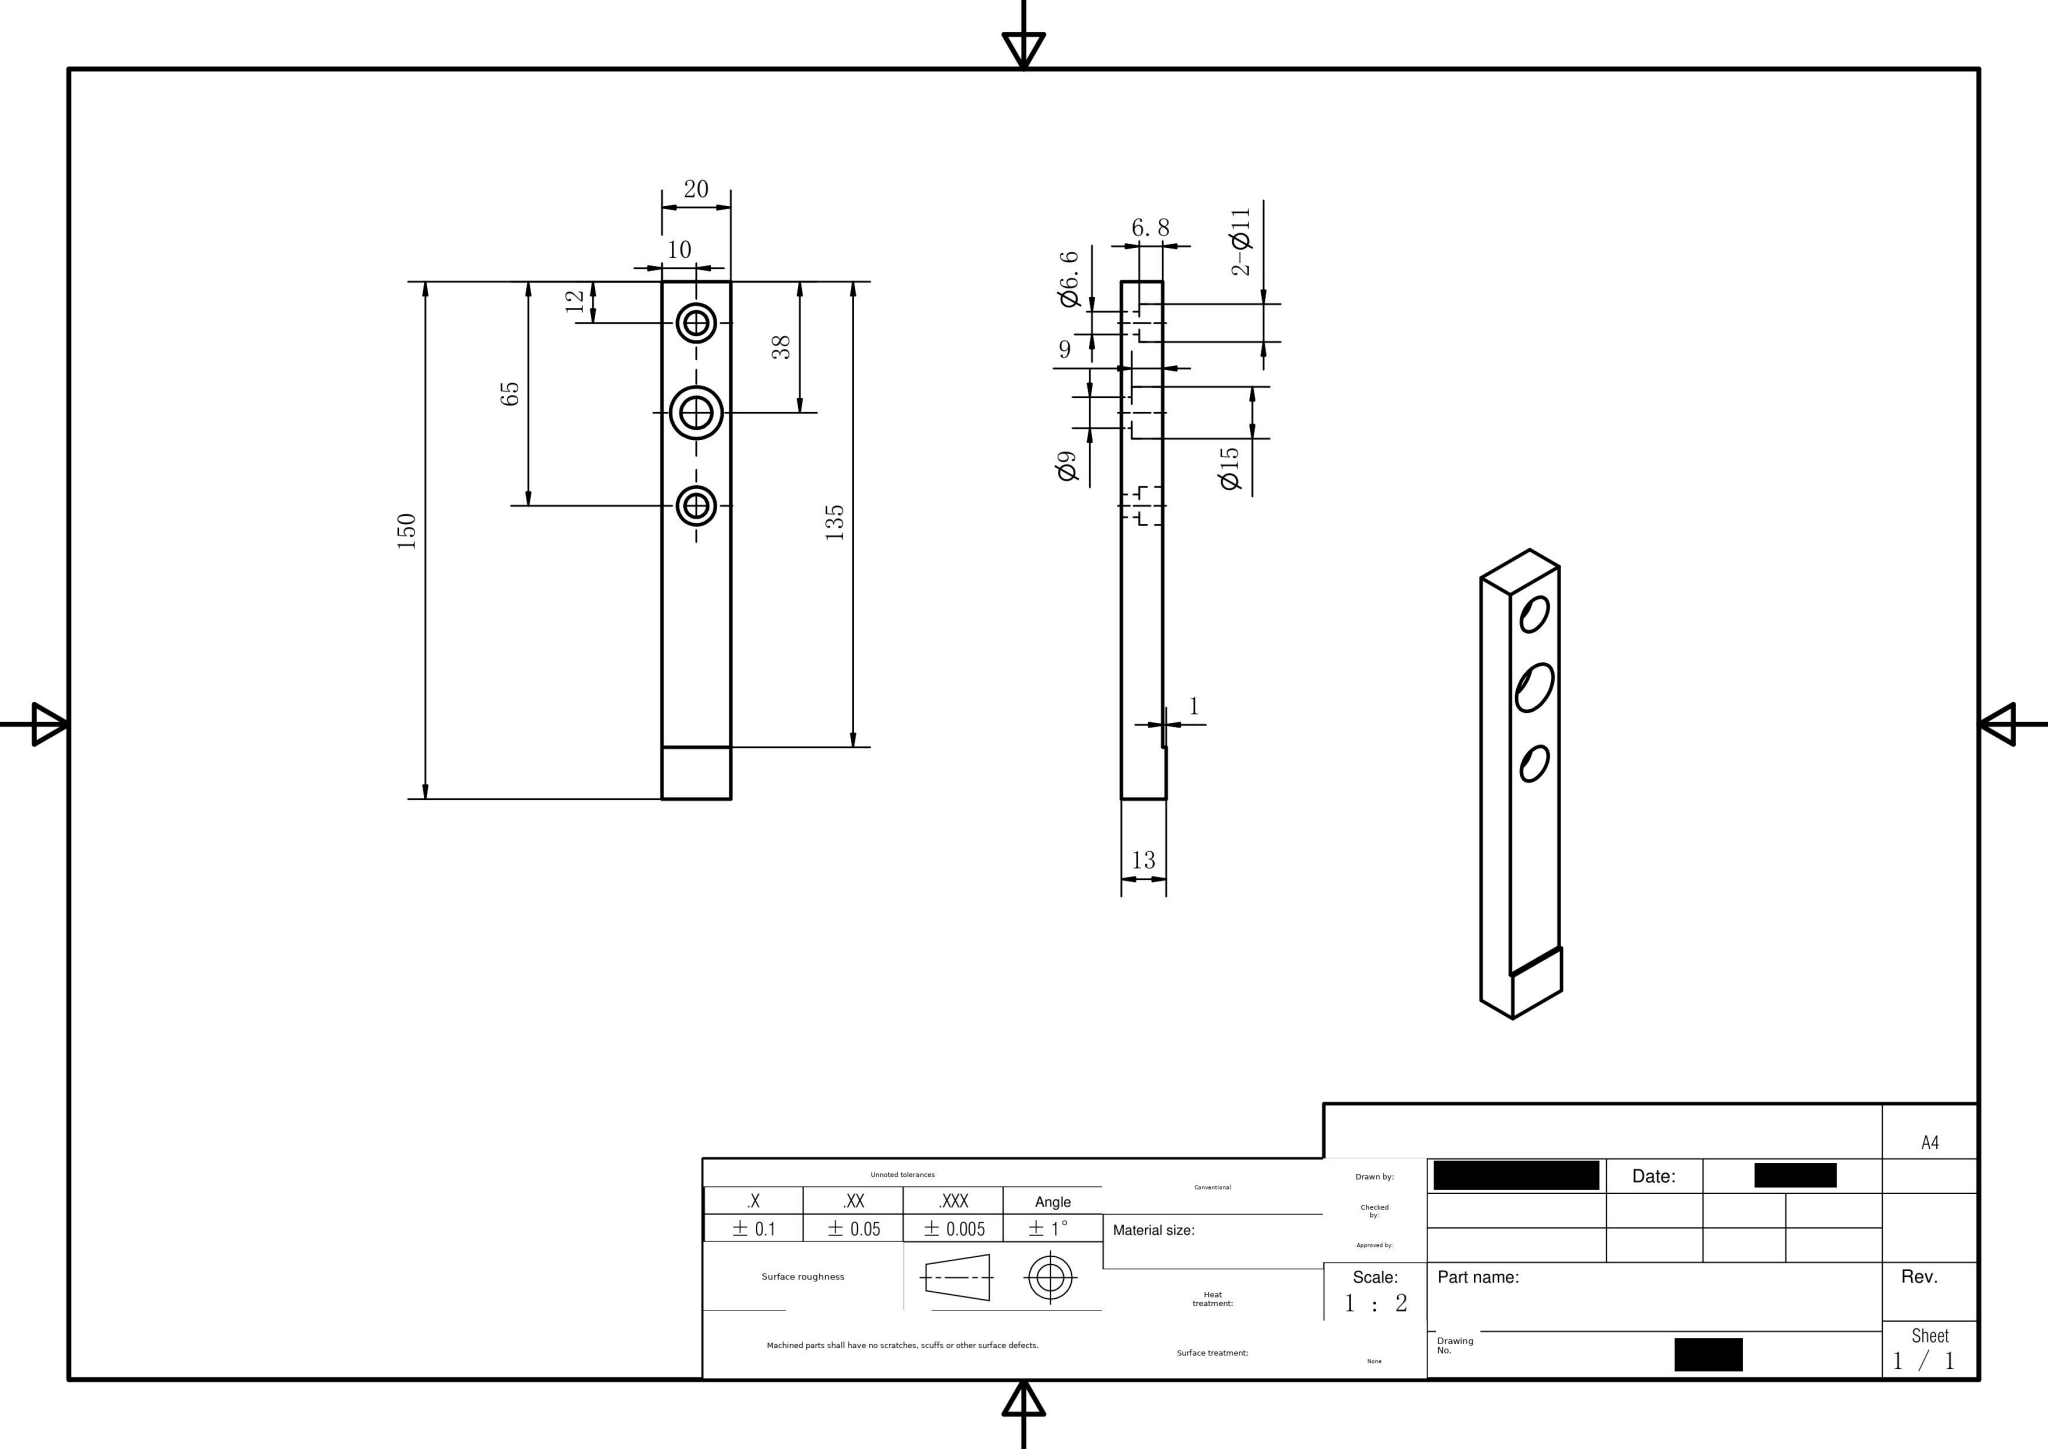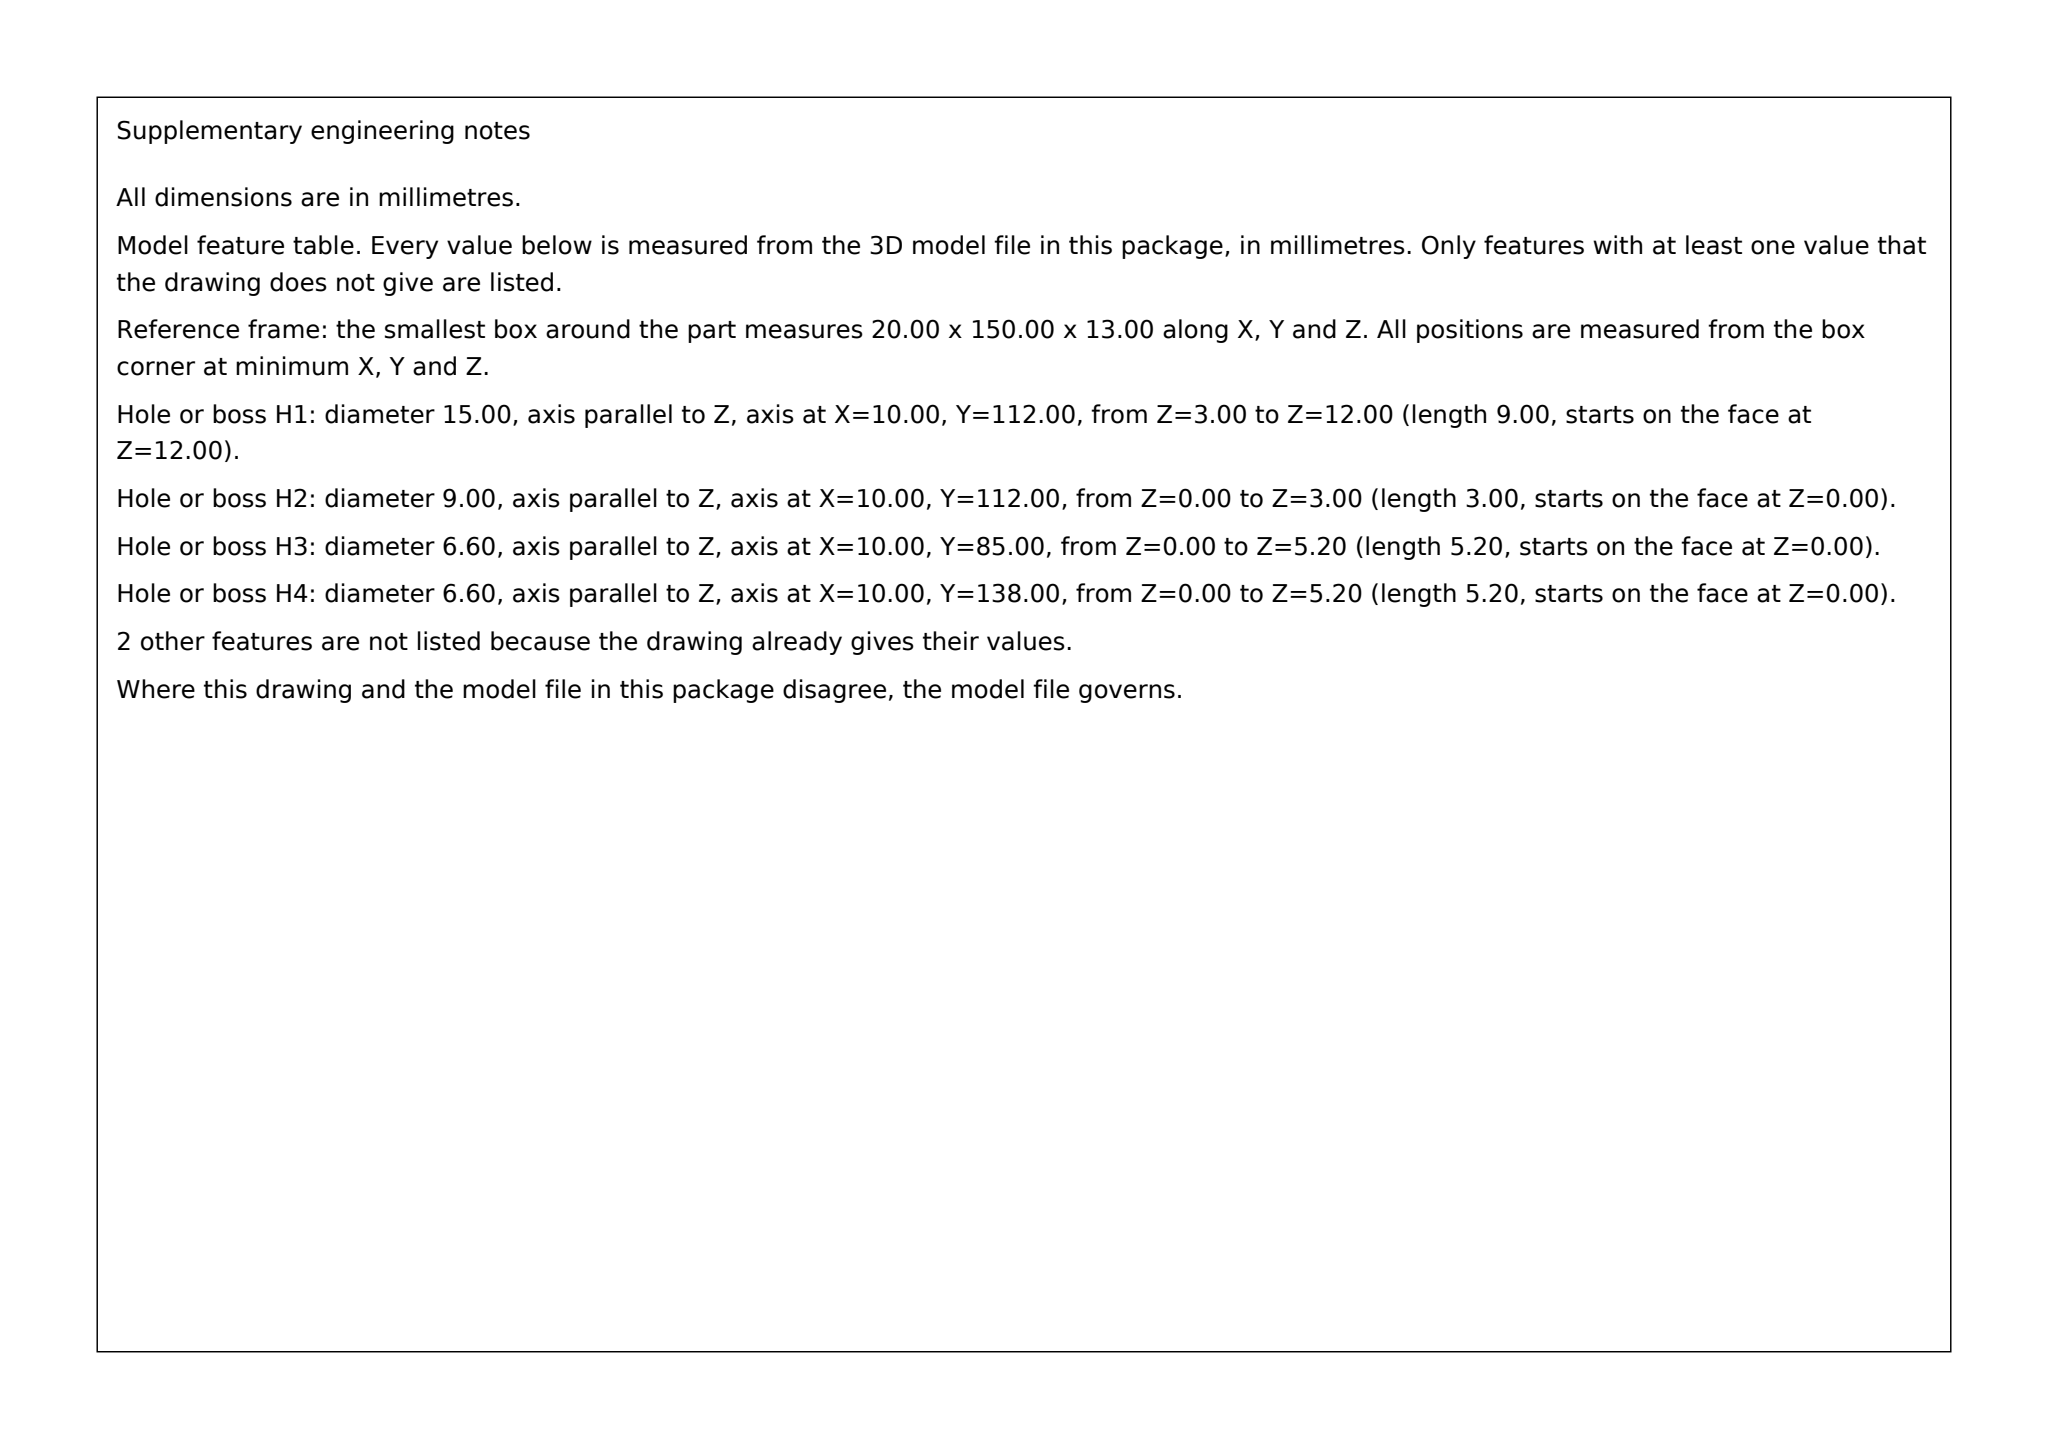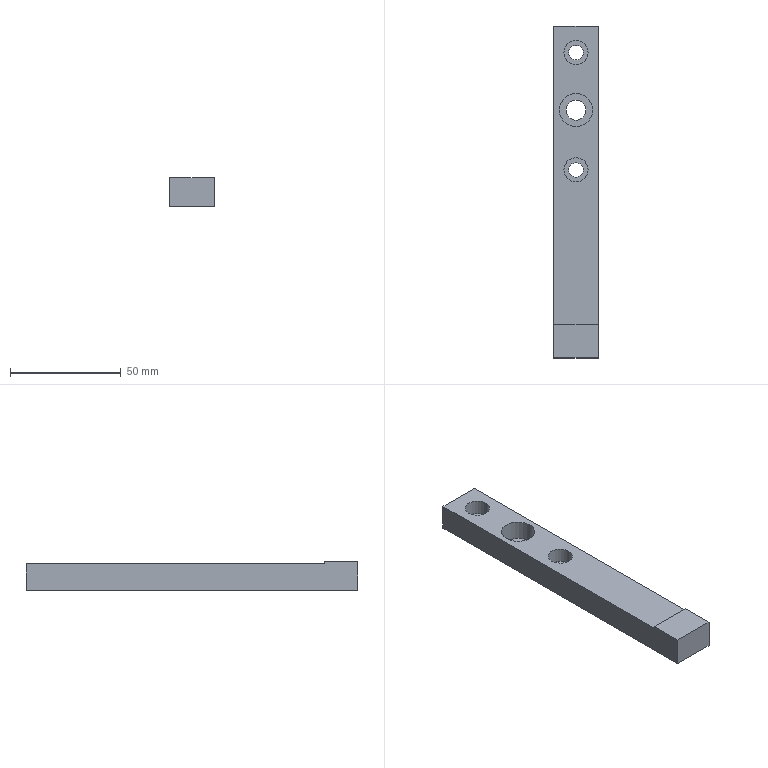Part | SolidWorks | mm | 1 solid | 23 faces | box 20 x 150 x 13 mm | volume 32870 mm3 | cylinder 12 | plane 11 | commonest cylinder face diameters 11 x4 6.6 x4 15 x2 9 x2
build123d program:
from build123d import *

# Parameters (mm, degrees)
SKETCH1_W                                  = 20
SKETCH1_H                                  = 150
BOSS_EXTRUDE1_DEPTH                        = 13
SKETCH2_W                                  = 1
SKETCH2_H                                  = 135
CUT_EXTRUDE1_DEPTH                         = 79.702
M6_HEX_HEAD_BOLT_COUNTERBORE_1_D           = 6.6
M6_HEX_HEAD_BOLT_COUNTERBORE_1_CBORE_D     = 11
M6_HEX_HEAD_BOLT_COUNTERBORE_1_CBORE_DEPTH = 6.8
M8_HEX_HEAD_BOLT_COUNTERBORE_1_D           = 9
M8_HEX_HEAD_BOLT_COUNTERBORE_1_CBORE_D     = 15
M8_HEX_HEAD_BOLT_COUNTERBORE_1_CBORE_DEPTH = 9


with BuildPart() as part:
    # Sketch1 → Boss-Extrude1 (new body)
    with BuildSketch(Plane.XY.offset(13)):
        Rectangle(SKETCH1_W, SKETCH1_H)
    extrude(amount=-BOSS_EXTRUDE1_DEPTH)

    # Sketch2 → Cut-Extrude1 (cut, through all)
    with BuildSketch(Plane(origin=(10, 0, 0), x_dir=(0, 0, -1), z_dir=(1, 0, 0))):
        with Locations((-12.5, 7.5)):
            Rectangle(SKETCH2_W, SKETCH2_H)
    extrude(amount=-CUT_EXTRUDE1_DEPTH, mode=Mode.SUBTRACT)

    # M6 Hex Head Bolt Counterbore 1 (through all)
    with Locations(Plane.XY.offset(12)):
        with Locations((0, 63), (0, 10)):
            CounterBoreHole(M6_HEX_HEAD_BOLT_COUNTERBORE_1_D / 2, M6_HEX_HEAD_BOLT_COUNTERBORE_1_CBORE_D / 2, M6_HEX_HEAD_BOLT_COUNTERBORE_1_CBORE_DEPTH)

    # M8 Hex Head Bolt Counterbore 1 (through all)
    with Locations(Plane.XY.offset(12)):
        with Locations((0, 37)):
            CounterBoreHole(M8_HEX_HEAD_BOLT_COUNTERBORE_1_D / 2, M8_HEX_HEAD_BOLT_COUNTERBORE_1_CBORE_D / 2, M8_HEX_HEAD_BOLT_COUNTERBORE_1_CBORE_DEPTH)


solid = part.part
STEP:
#1=CARTESIAN_POINT('',(-7.5,37.,3.));
#2=VERTEX_POINT('',#1);
#3=CARTESIAN_POINT('',(7.5,37.,3.));
#4=VERTEX_POINT('',#3);
#5=CARTESIAN_POINT('',(0.,37.,3.));
#6=DIRECTION('',(0.,0.,1.));
#7=DIRECTION('',(1.,0.,0.));
#8=AXIS2_PLACEMENT_3D('',#5,#6,#7);
#9=CIRCLE('',#8,7.5);
#10=EDGE_CURVE('',#2,#4,#9,.T.);
#11=ORIENTED_EDGE('',*,*,#10,.F.);
#12=CARTESIAN_POINT('',(-7.5,37.,12.));
#13=VERTEX_POINT('',#12);
#14=CARTESIAN_POINT('',(-7.5,37.,12.));
#15=DIRECTION('',(0.,0.,1.));
#16=VECTOR('',#15,1000.);
#17=LINE('',#14,#16);
#18=EDGE_CURVE('',#2,#13,#17,.T.);
#19=ORIENTED_EDGE('',*,*,#18,.T.);
#20=CARTESIAN_POINT('',(7.5,37.,12.));
#21=VERTEX_POINT('',#20);
#22=CARTESIAN_POINT('',(0.,37.,12.));
#23=DIRECTION('',(0.,0.,1.));
#24=DIRECTION('',(1.,0.,0.));
#25=AXIS2_PLACEMENT_3D('',#22,#23,#24);
#26=CIRCLE('',#25,7.5);
#27=EDGE_CURVE('',#13,#21,#26,.T.);
#28=ORIENTED_EDGE('',*,*,#27,.T.);
#29=CARTESIAN_POINT('',(7.5,37.,12.));
#30=DIRECTION('',(0.,0.,1.));
#31=VECTOR('',#30,1000.);
#32=LINE('',#29,#31);
#33=EDGE_CURVE('',#4,#21,#32,.T.);
#34=ORIENTED_EDGE('',*,*,#33,.F.);
#35=EDGE_LOOP('',(#11,#19,#28,#34));
#36=FACE_OUTER_BOUND('',#35,.T.);
#37=CARTESIAN_POINT('',(0.,37.,12.));
#38=DIRECTION('',(0.,0.,1.));
#39=DIRECTION('',(1.,0.,0.));
#40=AXIS2_PLACEMENT_3D('',#37,#38,#39);
#41=CYLINDRICAL_SURFACE('',#40,7.5);
#42=ADVANCED_FACE('',(#36),#41,.F.);
#43=CARTESIAN_POINT('',(-4.5,37.,0.));
#44=VERTEX_POINT('',#43);
#45=CARTESIAN_POINT('',(4.5,37.,0.));
#46=VERTEX_POINT('',#45);
#47=CARTESIAN_POINT('',(0.,37.,0.));
#48=DIRECTION('',(0.,0.,1.));
#49=DIRECTION('',(1.,0.,0.));
#50=AXIS2_PLACEMENT_3D('',#47,#48,#49);
#51=CIRCLE('',#50,4.5);
#52=EDGE_CURVE('',#44,#46,#51,.T.);
#53=ORIENTED_EDGE('',*,*,#52,.F.);
#54=CARTESIAN_POINT('',(-4.5,37.,3.));
#55=VERTEX_POINT('',#54);
#56=CARTESIAN_POINT('',(-4.5,37.,12.));
#57=DIRECTION('',(0.,0.,1.));
#58=VECTOR('',#57,1000.);
#59=LINE('',#56,#58);
#60=EDGE_CURVE('',#44,#55,#59,.T.);
#61=ORIENTED_EDGE('',*,*,#60,.T.);
#62=CARTESIAN_POINT('',(4.5,37.,3.));
#63=VERTEX_POINT('',#62);
#64=CARTESIAN_POINT('',(0.,37.,3.));
#65=DIRECTION('',(0.,0.,1.));
#66=DIRECTION('',(1.,0.,0.));
#67=AXIS2_PLACEMENT_3D('',#64,#65,#66);
#68=CIRCLE('',#67,4.5);
#69=EDGE_CURVE('',#55,#63,#68,.T.);
#70=ORIENTED_EDGE('',*,*,#69,.T.);
#71=CARTESIAN_POINT('',(4.5,37.,12.));
#72=DIRECTION('',(0.,0.,1.));
#73=VECTOR('',#72,1000.);
#74=LINE('',#71,#73);
#75=EDGE_CURVE('',#46,#63,#74,.T.);
#76=ORIENTED_EDGE('',*,*,#75,.F.);
#77=EDGE_LOOP('',(#53,#61,#70,#76));
#78=FACE_OUTER_BOUND('',#77,.T.);
#79=CARTESIAN_POINT('',(0.,37.,12.));
#80=DIRECTION('',(0.,0.,1.));
#81=DIRECTION('',(1.,0.,0.));
#82=AXIS2_PLACEMENT_3D('',#79,#80,#81);
#83=CYLINDRICAL_SURFACE('',#82,4.5);
#84=ADVANCED_FACE('',(#78),#83,.F.);
#85=CARTESIAN_POINT('',(-5.5,63.,5.2));
#86=VERTEX_POINT('',#85);
#87=CARTESIAN_POINT('',(5.5,63.,5.2));
#88=VERTEX_POINT('',#87);
#89=CARTESIAN_POINT('',(0.,63.,5.2));
#90=DIRECTION('',(0.,0.,1.));
#91=DIRECTION('',(1.,0.,0.));
#92=AXIS2_PLACEMENT_3D('',#89,#90,#91);
#93=CIRCLE('',#92,5.5);
#94=EDGE_CURVE('',#86,#88,#93,.T.);
#95=ORIENTED_EDGE('',*,*,#94,.F.);
#96=CARTESIAN_POINT('',(-5.5,63.,12.));
#97=VERTEX_POINT('',#96);
#98=CARTESIAN_POINT('',(-5.5,63.,12.));
#99=DIRECTION('',(0.,0.,1.));
#100=VECTOR('',#99,1000.);
#101=LINE('',#98,#100);
#102=EDGE_CURVE('',#86,#97,#101,.T.);
#103=ORIENTED_EDGE('',*,*,#102,.T.);
#104=CARTESIAN_POINT('',(5.5,63.,12.));
#105=VERTEX_POINT('',#104);
#106=CARTESIAN_POINT('',(0.,63.,12.));
#107=DIRECTION('',(0.,0.,1.));
#108=DIRECTION('',(1.,0.,0.));
#109=AXIS2_PLACEMENT_3D('',#106,#107,#108);
#110=CIRCLE('',#109,5.5);
#111=EDGE_CURVE('',#97,#105,#110,.T.);
#112=ORIENTED_EDGE('',*,*,#111,.T.);
#113=CARTESIAN_POINT('',(5.5,63.,12.));
#114=DIRECTION('',(0.,0.,1.));
#115=VECTOR('',#114,1000.);
#116=LINE('',#113,#115);
#117=EDGE_CURVE('',#88,#105,#116,.T.);
#118=ORIENTED_EDGE('',*,*,#117,.F.);
#119=EDGE_LOOP('',(#95,#103,#112,#118));
#120=FACE_OUTER_BOUND('',#119,.T.);
#121=CARTESIAN_POINT('',(0.,63.,12.));
#122=DIRECTION('',(0.,0.,1.));
#123=DIRECTION('',(1.,0.,0.));
#124=AXIS2_PLACEMENT_3D('',#121,#122,#123);
#125=CYLINDRICAL_SURFACE('',#124,5.5);
#126=ADVANCED_FACE('',(#120),#125,.F.);
#127=CARTESIAN_POINT('',(-3.3,63.,0.));
#128=VERTEX_POINT('',#127);
#129=CARTESIAN_POINT('',(3.3,63.,0.));
#130=VERTEX_POINT('',#129);
#131=CARTESIAN_POINT('',(0.,63.,0.));
#132=DIRECTION('',(0.,0.,1.));
#133=DIRECTION('',(1.,0.,0.));
#134=AXIS2_PLACEMENT_3D('',#131,#132,#133);
#135=CIRCLE('',#134,3.3);
#136=EDGE_CURVE('',#128,#130,#135,.T.);
#137=ORIENTED_EDGE('',*,*,#136,.F.);
#138=CARTESIAN_POINT('',(-3.3,63.,5.2));
#139=VERTEX_POINT('',#138);
#140=CARTESIAN_POINT('',(-3.3,63.,12.));
#141=DIRECTION('',(0.,0.,1.));
#142=VECTOR('',#141,1000.);
#143=LINE('',#140,#142);
#144=EDGE_CURVE('',#128,#139,#143,.T.);
#145=ORIENTED_EDGE('',*,*,#144,.T.);
#146=CARTESIAN_POINT('',(3.3,63.,5.2));
#147=VERTEX_POINT('',#146);
#148=CARTESIAN_POINT('',(0.,63.,5.2));
#149=DIRECTION('',(0.,0.,1.));
#150=DIRECTION('',(1.,0.,0.));
#151=AXIS2_PLACEMENT_3D('',#148,#149,#150);
#152=CIRCLE('',#151,3.3);
#153=EDGE_CURVE('',#139,#147,#152,.T.);
#154=ORIENTED_EDGE('',*,*,#153,.T.);
#155=CARTESIAN_POINT('',(3.3,63.,12.));
#156=DIRECTION('',(0.,0.,1.));
#157=VECTOR('',#156,1000.);
#158=LINE('',#155,#157);
#159=EDGE_CURVE('',#130,#147,#158,.T.);
#160=ORIENTED_EDGE('',*,*,#159,.F.);
#161=EDGE_LOOP('',(#137,#145,#154,#160));
#162=FACE_OUTER_BOUND('',#161,.T.);
#163=CARTESIAN_POINT('',(0.,63.,12.));
#164=DIRECTION('',(0.,0.,1.));
#165=DIRECTION('',(1.,0.,0.));
#166=AXIS2_PLACEMENT_3D('',#163,#164,#165);
#167=CYLINDRICAL_SURFACE('',#166,3.3);
#168=ADVANCED_FACE('',(#162),#167,.F.);
#169=CARTESIAN_POINT('',(-5.5,10.,5.2));
#170=VERTEX_POINT('',#169);
#171=CARTESIAN_POINT('',(5.5,10.,5.2));
#172=VERTEX_POINT('',#171);
#173=CARTESIAN_POINT('',(0.,10.,5.2));
#174=DIRECTION('',(0.,0.,1.));
#175=DIRECTION('',(1.,0.,0.));
#176=AXIS2_PLACEMENT_3D('',#173,#174,#175);
#177=CIRCLE('',#176,5.5);
#178=EDGE_CURVE('',#170,#172,#177,.T.);
#179=ORIENTED_EDGE('',*,*,#178,.F.);
#180=CARTESIAN_POINT('',(-5.5,10.,12.));
#181=VERTEX_POINT('',#180);
#182=CARTESIAN_POINT('',(-5.5,10.,12.));
#183=DIRECTION('',(0.,0.,1.));
#184=VECTOR('',#183,1000.);
#185=LINE('',#182,#184);
#186=EDGE_CURVE('',#170,#181,#185,.T.);
#187=ORIENTED_EDGE('',*,*,#186,.T.);
#188=CARTESIAN_POINT('',(5.5,10.,12.));
#189=VERTEX_POINT('',#188);
#190=CARTESIAN_POINT('',(0.,10.,12.));
#191=DIRECTION('',(0.,0.,1.));
#192=DIRECTION('',(1.,0.,0.));
#193=AXIS2_PLACEMENT_3D('',#190,#191,#192);
#194=CIRCLE('',#193,5.5);
#195=EDGE_CURVE('',#181,#189,#194,.T.);
#196=ORIENTED_EDGE('',*,*,#195,.T.);
#197=CARTESIAN_POINT('',(5.5,10.,12.));
#198=DIRECTION('',(0.,0.,1.));
#199=VECTOR('',#198,1000.);
#200=LINE('',#197,#199);
#201=EDGE_CURVE('',#172,#189,#200,.T.);
#202=ORIENTED_EDGE('',*,*,#201,.F.);
#203=EDGE_LOOP('',(#179,#187,#196,#202));
#204=FACE_OUTER_BOUND('',#203,.T.);
#205=CARTESIAN_POINT('',(0.,10.,12.));
#206=DIRECTION('',(0.,0.,1.));
#207=DIRECTION('',(1.,0.,0.));
#208=AXIS2_PLACEMENT_3D('',#205,#206,#207);
#209=CYLINDRICAL_SURFACE('',#208,5.5);
#210=ADVANCED_FACE('',(#204),#209,.F.);
#211=CARTESIAN_POINT('',(-3.3,10.,0.));
#212=VERTEX_POINT('',#211);
#213=CARTESIAN_POINT('',(3.3,10.,0.));
#214=VERTEX_POINT('',#213);
#215=CARTESIAN_POINT('',(0.,10.,0.));
#216=DIRECTION('',(0.,0.,1.));
#217=DIRECTION('',(1.,0.,0.));
#218=AXIS2_PLACEMENT_3D('',#215,#216,#217);
#219=CIRCLE('',#218,3.3);
#220=EDGE_CURVE('',#212,#214,#219,.T.);
#221=ORIENTED_EDGE('',*,*,#220,.F.);
#222=CARTESIAN_POINT('',(-3.3,10.,5.2));
#223=VERTEX_POINT('',#222);
#224=CARTESIAN_POINT('',(-3.3,10.,12.));
#225=DIRECTION('',(0.,0.,1.));
#226=VECTOR('',#225,1000.);
#227=LINE('',#224,#226);
#228=EDGE_CURVE('',#212,#223,#227,.T.);
#229=ORIENTED_EDGE('',*,*,#228,.T.);
#230=CARTESIAN_POINT('',(3.3,10.,5.2));
#231=VERTEX_POINT('',#230);
#232=CARTESIAN_POINT('',(0.,10.,5.2));
#233=DIRECTION('',(0.,0.,1.));
#234=DIRECTION('',(1.,0.,0.));
#235=AXIS2_PLACEMENT_3D('',#232,#233,#234);
#236=CIRCLE('',#235,3.3);
#237=EDGE_CURVE('',#223,#231,#236,.T.);
#238=ORIENTED_EDGE('',*,*,#237,.T.);
#239=CARTESIAN_POINT('',(3.3,10.,12.));
#240=DIRECTION('',(0.,0.,1.));
#241=VECTOR('',#240,1000.);
#242=LINE('',#239,#241);
#243=EDGE_CURVE('',#214,#231,#242,.T.);
#244=ORIENTED_EDGE('',*,*,#243,.F.);
#245=EDGE_LOOP('',(#221,#229,#238,#244));
#246=FACE_OUTER_BOUND('',#245,.T.);
#247=CARTESIAN_POINT('',(0.,10.,12.));
#248=DIRECTION('',(0.,0.,1.));
#249=DIRECTION('',(1.,0.,0.));
#250=AXIS2_PLACEMENT_3D('',#247,#248,#249);
#251=CYLINDRICAL_SURFACE('',#250,3.3);
#252=ADVANCED_FACE('',(#246),#251,.F.);
#253=CARTESIAN_POINT('',(-10.,75.,12.));
#254=VERTEX_POINT('',#253);
#255=CARTESIAN_POINT('',(10.,75.,12.));
#256=VERTEX_POINT('',#255);
#257=CARTESIAN_POINT('',(-10.,75.,12.));
#258=DIRECTION('',(1.,-0.,0.));
#259=VECTOR('',#258,1000.);
#260=LINE('',#257,#259);
#261=EDGE_CURVE('',#254,#256,#260,.T.);
#262=ORIENTED_EDGE('',*,*,#261,.T.);
#263=CARTESIAN_POINT('',(10.,75.,0.));
#264=VERTEX_POINT('',#263);
#265=CARTESIAN_POINT('',(10.,75.,0.));
#266=DIRECTION('',(0.,0.,1.));
#267=VECTOR('',#266,1000.);
#268=LINE('',#265,#267);
#269=EDGE_CURVE('',#264,#256,#268,.T.);
#270=ORIENTED_EDGE('',*,*,#269,.F.);
#271=CARTESIAN_POINT('',(-10.,75.,0.));
#272=VERTEX_POINT('',#271);
#273=CARTESIAN_POINT('',(10.,75.,0.));
#274=DIRECTION('',(-1.,0.,0.));
#275=VECTOR('',#274,1000.);
#276=LINE('',#273,#275);
#277=EDGE_CURVE('',#264,#272,#276,.T.);
#278=ORIENTED_EDGE('',*,*,#277,.T.);
#279=CARTESIAN_POINT('',(-10.,75.,0.));
#280=DIRECTION('',(0.,0.,1.));
#281=VECTOR('',#280,1000.);
#282=LINE('',#279,#281);
#283=EDGE_CURVE('',#272,#254,#282,.T.);
#284=ORIENTED_EDGE('',*,*,#283,.T.);
#285=EDGE_LOOP('',(#262,#270,#278,#284));
#286=FACE_OUTER_BOUND('',#285,.T.);
#287=CARTESIAN_POINT('',(10.,75.,0.));
#288=DIRECTION('',(0.,1.,0.));
#289=DIRECTION('',(-1.,0.,0.));
#290=AXIS2_PLACEMENT_3D('',#287,#288,#289);
#291=PLANE('',#290);
#292=ADVANCED_FACE('',(#286),#291,.T.);
#293=CARTESIAN_POINT('',(10.,-60.,12.));
#294=VERTEX_POINT('',#293);
#295=CARTESIAN_POINT('',(10.,-60.,12.));
#296=DIRECTION('',(0.,1.,0.));
#297=VECTOR('',#296,1000.);
#298=LINE('',#295,#297);
#299=EDGE_CURVE('',#294,#256,#298,.T.);
#300=ORIENTED_EDGE('',*,*,#299,.F.);
#301=CARTESIAN_POINT('',(10.,-60.,13.));
#302=VERTEX_POINT('',#301);
#303=CARTESIAN_POINT('',(10.,-60.,13.));
#304=DIRECTION('',(0.,0.,-1.));
#305=VECTOR('',#304,1000.);
#306=LINE('',#303,#305);
#307=EDGE_CURVE('',#302,#294,#306,.T.);
#308=ORIENTED_EDGE('',*,*,#307,.F.);
#309=CARTESIAN_POINT('',(10.,-75.,13.));
#310=VERTEX_POINT('',#309);
#311=CARTESIAN_POINT('',(10.,-75.,13.));
#312=DIRECTION('',(0.,1.,0.));
#313=VECTOR('',#312,1000.);
#314=LINE('',#311,#313);
#315=EDGE_CURVE('',#310,#302,#314,.T.);
#316=ORIENTED_EDGE('',*,*,#315,.F.);
#317=CARTESIAN_POINT('',(10.,-75.,0.));
#318=VERTEX_POINT('',#317);
#319=CARTESIAN_POINT('',(10.,-75.,0.));
#320=DIRECTION('',(0.,0.,1.));
#321=VECTOR('',#320,1000.);
#322=LINE('',#319,#321);
#323=EDGE_CURVE('',#318,#310,#322,.T.);
#324=ORIENTED_EDGE('',*,*,#323,.F.);
#325=CARTESIAN_POINT('',(10.,-75.,0.));
#326=DIRECTION('',(0.,1.,0.));
#327=VECTOR('',#326,1000.);
#328=LINE('',#325,#327);
#329=EDGE_CURVE('',#318,#264,#328,.T.);
#330=ORIENTED_EDGE('',*,*,#329,.T.);
#331=ORIENTED_EDGE('',*,*,#269,.T.);
#332=EDGE_LOOP('',(#300,#308,#316,#324,#330,#331));
#333=FACE_OUTER_BOUND('',#332,.T.);
#334=CARTESIAN_POINT('',(10.,-75.,0.));
#335=DIRECTION('',(1.,-0.,0.));
#336=DIRECTION('',(0.,1.,0.));
#337=AXIS2_PLACEMENT_3D('',#334,#335,#336);
#338=PLANE('',#337);
#339=ADVANCED_FACE('',(#333),#338,.T.);
#340=CARTESIAN_POINT('',(-10.,-75.,13.));
#341=VERTEX_POINT('',#340);
#342=CARTESIAN_POINT('',(-10.,-75.,13.));
#343=DIRECTION('',(1.,0.,0.));
#344=VECTOR('',#343,1000.);
#345=LINE('',#342,#344);
#346=EDGE_CURVE('',#341,#310,#345,.T.);
#347=ORIENTED_EDGE('',*,*,#346,.F.);
#348=CARTESIAN_POINT('',(-10.,-75.,0.));
#349=VERTEX_POINT('',#348);
#350=CARTESIAN_POINT('',(-10.,-75.,0.));
#351=DIRECTION('',(0.,0.,1.));
#352=VECTOR('',#351,1000.);
#353=LINE('',#350,#352);
#354=EDGE_CURVE('',#349,#341,#353,.T.);
#355=ORIENTED_EDGE('',*,*,#354,.F.);
#356=CARTESIAN_POINT('',(-10.,-75.,0.));
#357=DIRECTION('',(1.,0.,0.));
#358=VECTOR('',#357,1000.);
#359=LINE('',#356,#358);
#360=EDGE_CURVE('',#349,#318,#359,.T.);
#361=ORIENTED_EDGE('',*,*,#360,.T.);
#362=ORIENTED_EDGE('',*,*,#323,.T.);
#363=EDGE_LOOP('',(#347,#355,#361,#362));
#364=FACE_OUTER_BOUND('',#363,.T.);
#365=CARTESIAN_POINT('',(-10.,-75.,0.));
#366=DIRECTION('',(0.,-1.,0.));
#367=DIRECTION('',(0.,0.,-1.));
#368=AXIS2_PLACEMENT_3D('',#365,#366,#367);
#369=PLANE('',#368);
#370=ADVANCED_FACE('',(#364),#369,.T.);
#371=CARTESIAN_POINT('',(-10.,-60.,12.));
#372=VERTEX_POINT('',#371);
#373=CARTESIAN_POINT('',(-10.,-60.,12.));
#374=DIRECTION('',(0.,1.,0.));
#375=VECTOR('',#374,1000.);
#376=LINE('',#373,#375);
#377=EDGE_CURVE('',#372,#254,#376,.T.);
#378=ORIENTED_EDGE('',*,*,#377,.T.);
#379=ORIENTED_EDGE('',*,*,#283,.F.);
#380=CARTESIAN_POINT('',(-10.,75.,0.));
#381=DIRECTION('',(0.,-1.,0.));
#382=VECTOR('',#381,1000.);
#383=LINE('',#380,#382);
#384=EDGE_CURVE('',#272,#349,#383,.T.);
#385=ORIENTED_EDGE('',*,*,#384,.T.);
#386=ORIENTED_EDGE('',*,*,#354,.T.);
#387=CARTESIAN_POINT('',(-10.,-60.,13.));
#388=VERTEX_POINT('',#387);
#389=CARTESIAN_POINT('',(-10.,75.,13.));
#390=DIRECTION('',(0.,-1.,0.));
#391=VECTOR('',#390,1000.);
#392=LINE('',#389,#391);
#393=EDGE_CURVE('',#388,#341,#392,.T.);
#394=ORIENTED_EDGE('',*,*,#393,.F.);
#395=CARTESIAN_POINT('',(-10.,-60.,13.));
#396=DIRECTION('',(0.,0.,-1.));
#397=VECTOR('',#396,1000.);
#398=LINE('',#395,#397);
#399=EDGE_CURVE('',#388,#372,#398,.T.);
#400=ORIENTED_EDGE('',*,*,#399,.T.);
#401=EDGE_LOOP('',(#378,#379,#385,#386,#394,#400));
#402=FACE_OUTER_BOUND('',#401,.T.);
#403=CARTESIAN_POINT('',(-10.,75.,0.));
#404=DIRECTION('',(-1.,-0.,0.));
#405=DIRECTION('',(0.,-1.,0.));
#406=AXIS2_PLACEMENT_3D('',#403,#404,#405);
#407=PLANE('',#406);
#408=ADVANCED_FACE('',(#402),#407,.T.);
#409=CARTESIAN_POINT('',(0.,37.,0.));
#410=DIRECTION('',(0.,0.,1.));
#411=DIRECTION('',(1.,0.,0.));
#412=AXIS2_PLACEMENT_3D('',#409,#410,#411);
#413=CIRCLE('',#412,4.5);
#414=EDGE_CURVE('',#46,#44,#413,.T.);
#415=ORIENTED_EDGE('',*,*,#414,.T.);
#416=ORIENTED_EDGE('',*,*,#52,.T.);
#417=EDGE_LOOP('',(#415,#416));
#418=FACE_BOUND('',#417,.T.);
#419=CARTESIAN_POINT('',(0.,63.,0.));
#420=DIRECTION('',(0.,0.,1.));
#421=DIRECTION('',(1.,0.,0.));
#422=AXIS2_PLACEMENT_3D('',#419,#420,#421);
#423=CIRCLE('',#422,3.3);
#424=EDGE_CURVE('',#130,#128,#423,.T.);
#425=ORIENTED_EDGE('',*,*,#424,.T.);
#426=ORIENTED_EDGE('',*,*,#136,.T.);
#427=EDGE_LOOP('',(#425,#426));
#428=FACE_BOUND('',#427,.T.);
#429=CARTESIAN_POINT('',(0.,10.,0.));
#430=DIRECTION('',(0.,0.,1.));
#431=DIRECTION('',(1.,0.,0.));
#432=AXIS2_PLACEMENT_3D('',#429,#430,#431);
#433=CIRCLE('',#432,3.3);
#434=EDGE_CURVE('',#214,#212,#433,.T.);
#435=ORIENTED_EDGE('',*,*,#434,.T.);
#436=ORIENTED_EDGE('',*,*,#220,.T.);
#437=EDGE_LOOP('',(#435,#436));
#438=FACE_BOUND('',#437,.T.);
#439=ORIENTED_EDGE('',*,*,#277,.F.);
#440=ORIENTED_EDGE('',*,*,#329,.F.);
#441=ORIENTED_EDGE('',*,*,#360,.F.);
#442=ORIENTED_EDGE('',*,*,#384,.F.);
#443=EDGE_LOOP('',(#439,#440,#441,#442));
#444=FACE_OUTER_BOUND('',#443,.T.);
#445=CARTESIAN_POINT('',(0.,0.,0.));
#446=DIRECTION('',(0.,0.,1.));
#447=DIRECTION('',(1.,0.,0.));
#448=AXIS2_PLACEMENT_3D('',#445,#446,#447);
#449=PLANE('',#448);
#450=ADVANCED_FACE('',(#418,#428,#438,#444),#449,.F.);
#451=CARTESIAN_POINT('',(-10.,-60.,13.));
#452=DIRECTION('',(1.,-0.,0.));
#453=VECTOR('',#452,1000.);
#454=LINE('',#451,#453);
#455=EDGE_CURVE('',#388,#302,#454,.T.);
#456=ORIENTED_EDGE('',*,*,#455,.F.);
#457=ORIENTED_EDGE('',*,*,#393,.T.);
#458=ORIENTED_EDGE('',*,*,#346,.T.);
#459=ORIENTED_EDGE('',*,*,#315,.T.);
#460=EDGE_LOOP('',(#456,#457,#458,#459));
#461=FACE_OUTER_BOUND('',#460,.T.);
#462=CARTESIAN_POINT('',(0.,0.,13.));
#463=DIRECTION('',(0.,0.,1.));
#464=DIRECTION('',(1.,0.,0.));
#465=AXIS2_PLACEMENT_3D('',#462,#463,#464);
#466=PLANE('',#465);
#467=ADVANCED_FACE('',(#461),#466,.T.);
#468=CARTESIAN_POINT('',(0.,37.,12.));
#469=DIRECTION('',(0.,0.,1.));
#470=DIRECTION('',(1.,0.,0.));
#471=AXIS2_PLACEMENT_3D('',#468,#469,#470);
#472=CIRCLE('',#471,7.5);
#473=EDGE_CURVE('',#21,#13,#472,.T.);
#474=ORIENTED_EDGE('',*,*,#473,.F.);
#475=ORIENTED_EDGE('',*,*,#27,.F.);
#476=EDGE_LOOP('',(#474,#475));
#477=FACE_BOUND('',#476,.T.);
#478=CARTESIAN_POINT('',(0.,63.,12.));
#479=DIRECTION('',(0.,0.,1.));
#480=DIRECTION('',(1.,0.,0.));
#481=AXIS2_PLACEMENT_3D('',#478,#479,#480);
#482=CIRCLE('',#481,5.5);
#483=EDGE_CURVE('',#105,#97,#482,.T.);
#484=ORIENTED_EDGE('',*,*,#483,.F.);
#485=ORIENTED_EDGE('',*,*,#111,.F.);
#486=EDGE_LOOP('',(#484,#485));
#487=FACE_BOUND('',#486,.T.);
#488=CARTESIAN_POINT('',(0.,10.,12.));
#489=DIRECTION('',(0.,0.,1.));
#490=DIRECTION('',(1.,0.,0.));
#491=AXIS2_PLACEMENT_3D('',#488,#489,#490);
#492=CIRCLE('',#491,5.5);
#493=EDGE_CURVE('',#189,#181,#492,.T.);
#494=ORIENTED_EDGE('',*,*,#493,.F.);
#495=ORIENTED_EDGE('',*,*,#195,.F.);
#496=EDGE_LOOP('',(#494,#495));
#497=FACE_BOUND('',#496,.T.);
#498=ORIENTED_EDGE('',*,*,#299,.T.);
#499=ORIENTED_EDGE('',*,*,#261,.F.);
#500=ORIENTED_EDGE('',*,*,#377,.F.);
#501=CARTESIAN_POINT('',(-10.,-60.,12.));
#502=DIRECTION('',(1.,-0.,0.));
#503=VECTOR('',#502,1000.);
#504=LINE('',#501,#503);
#505=EDGE_CURVE('',#372,#294,#504,.T.);
#506=ORIENTED_EDGE('',*,*,#505,.T.);
#507=EDGE_LOOP('',(#498,#499,#500,#506));
#508=FACE_OUTER_BOUND('',#507,.T.);
#509=CARTESIAN_POINT('',(-10.,-60.,12.));
#510=DIRECTION('',(0.,0.,-1.));
#511=DIRECTION('',(-1.,0.,0.));
#512=AXIS2_PLACEMENT_3D('',#509,#510,#511);
#513=PLANE('',#512);
#514=ADVANCED_FACE('',(#477,#487,#497,#508),#513,.F.);
#515=ORIENTED_EDGE('',*,*,#307,.T.);
#516=ORIENTED_EDGE('',*,*,#505,.F.);
#517=ORIENTED_EDGE('',*,*,#399,.F.);
#518=ORIENTED_EDGE('',*,*,#455,.T.);
#519=EDGE_LOOP('',(#515,#516,#517,#518));
#520=FACE_OUTER_BOUND('',#519,.T.);
#521=CARTESIAN_POINT('',(-10.,-60.,13.));
#522=DIRECTION('',(-0.,-1.,0.));
#523=DIRECTION('',(1.,-0.,0.));
#524=AXIS2_PLACEMENT_3D('',#521,#522,#523);
#525=PLANE('',#524);
#526=ADVANCED_FACE('',(#520),#525,.F.);
#527=ORIENTED_EDGE('',*,*,#228,.F.);
#528=ORIENTED_EDGE('',*,*,#434,.F.);
#529=ORIENTED_EDGE('',*,*,#243,.T.);
#530=CARTESIAN_POINT('',(0.,10.,5.2));
#531=DIRECTION('',(0.,0.,1.));
#532=DIRECTION('',(1.,0.,0.));
#533=AXIS2_PLACEMENT_3D('',#530,#531,#532);
#534=CIRCLE('',#533,3.3);
#535=EDGE_CURVE('',#231,#223,#534,.T.);
#536=ORIENTED_EDGE('',*,*,#535,.T.);
#537=EDGE_LOOP('',(#527,#528,#529,#536));
#538=FACE_OUTER_BOUND('',#537,.T.);
#539=CARTESIAN_POINT('',(0.,10.,12.));
#540=DIRECTION('',(0.,0.,1.));
#541=DIRECTION('',(1.,0.,0.));
#542=AXIS2_PLACEMENT_3D('',#539,#540,#541);
#543=CYLINDRICAL_SURFACE('',#542,3.3);
#544=ADVANCED_FACE('',(#538),#543,.F.);
#545=ORIENTED_EDGE('',*,*,#535,.F.);
#546=ORIENTED_EDGE('',*,*,#237,.F.);
#547=EDGE_LOOP('',(#545,#546));
#548=FACE_BOUND('',#547,.T.);
#549=CARTESIAN_POINT('',(0.,10.,5.2));
#550=DIRECTION('',(0.,0.,1.));
#551=DIRECTION('',(1.,0.,0.));
#552=AXIS2_PLACEMENT_3D('',#549,#550,#551);
#553=CIRCLE('',#552,5.5);
#554=EDGE_CURVE('',#172,#170,#553,.T.);
#555=ORIENTED_EDGE('',*,*,#554,.T.);
#556=ORIENTED_EDGE('',*,*,#178,.T.);
#557=EDGE_LOOP('',(#555,#556));
#558=FACE_OUTER_BOUND('',#557,.T.);
#559=CARTESIAN_POINT('',(3.3,10.,5.2));
#560=DIRECTION('',(0.,0.,-1.));
#561=DIRECTION('',(-1.,0.,0.));
#562=AXIS2_PLACEMENT_3D('',#559,#560,#561);
#563=PLANE('',#562);
#564=ADVANCED_FACE('',(#548,#558),#563,.F.);
#565=ORIENTED_EDGE('',*,*,#186,.F.);
#566=ORIENTED_EDGE('',*,*,#554,.F.);
#567=ORIENTED_EDGE('',*,*,#201,.T.);
#568=ORIENTED_EDGE('',*,*,#493,.T.);
#569=EDGE_LOOP('',(#565,#566,#567,#568));
#570=FACE_OUTER_BOUND('',#569,.T.);
#571=CARTESIAN_POINT('',(0.,10.,12.));
#572=DIRECTION('',(0.,0.,1.));
#573=DIRECTION('',(1.,0.,0.));
#574=AXIS2_PLACEMENT_3D('',#571,#572,#573);
#575=CYLINDRICAL_SURFACE('',#574,5.5);
#576=ADVANCED_FACE('',(#570),#575,.F.);
#577=ORIENTED_EDGE('',*,*,#144,.F.);
#578=ORIENTED_EDGE('',*,*,#424,.F.);
#579=ORIENTED_EDGE('',*,*,#159,.T.);
#580=CARTESIAN_POINT('',(0.,63.,5.2));
#581=DIRECTION('',(0.,0.,1.));
#582=DIRECTION('',(1.,0.,0.));
#583=AXIS2_PLACEMENT_3D('',#580,#581,#582);
#584=CIRCLE('',#583,3.3);
#585=EDGE_CURVE('',#147,#139,#584,.T.);
#586=ORIENTED_EDGE('',*,*,#585,.T.);
#587=EDGE_LOOP('',(#577,#578,#579,#586));
#588=FACE_OUTER_BOUND('',#587,.T.);
#589=CARTESIAN_POINT('',(0.,63.,12.));
#590=DIRECTION('',(0.,0.,1.));
#591=DIRECTION('',(1.,0.,0.));
#592=AXIS2_PLACEMENT_3D('',#589,#590,#591);
#593=CYLINDRICAL_SURFACE('',#592,3.3);
#594=ADVANCED_FACE('',(#588),#593,.F.);
#595=ORIENTED_EDGE('',*,*,#585,.F.);
#596=ORIENTED_EDGE('',*,*,#153,.F.);
#597=EDGE_LOOP('',(#595,#596));
#598=FACE_BOUND('',#597,.T.);
#599=CARTESIAN_POINT('',(0.,63.,5.2));
#600=DIRECTION('',(0.,0.,1.));
#601=DIRECTION('',(1.,0.,0.));
#602=AXIS2_PLACEMENT_3D('',#599,#600,#601);
#603=CIRCLE('',#602,5.5);
#604=EDGE_CURVE('',#88,#86,#603,.T.);
#605=ORIENTED_EDGE('',*,*,#604,.T.);
#606=ORIENTED_EDGE('',*,*,#94,.T.);
#607=EDGE_LOOP('',(#605,#606));
#608=FACE_OUTER_BOUND('',#607,.T.);
#609=CARTESIAN_POINT('',(3.3,63.,5.2));
#610=DIRECTION('',(0.,0.,-1.));
#611=DIRECTION('',(-1.,0.,0.));
#612=AXIS2_PLACEMENT_3D('',#609,#610,#611);
#613=PLANE('',#612);
#614=ADVANCED_FACE('',(#598,#608),#613,.F.);
#615=ORIENTED_EDGE('',*,*,#102,.F.);
#616=ORIENTED_EDGE('',*,*,#604,.F.);
#617=ORIENTED_EDGE('',*,*,#117,.T.);
#618=ORIENTED_EDGE('',*,*,#483,.T.);
#619=EDGE_LOOP('',(#615,#616,#617,#618));
#620=FACE_OUTER_BOUND('',#619,.T.);
#621=CARTESIAN_POINT('',(0.,63.,12.));
#622=DIRECTION('',(0.,0.,1.));
#623=DIRECTION('',(1.,0.,0.));
#624=AXIS2_PLACEMENT_3D('',#621,#622,#623);
#625=CYLINDRICAL_SURFACE('',#624,5.5);
#626=ADVANCED_FACE('',(#620),#625,.F.);
#627=ORIENTED_EDGE('',*,*,#60,.F.);
#628=ORIENTED_EDGE('',*,*,#414,.F.);
#629=ORIENTED_EDGE('',*,*,#75,.T.);
#630=CARTESIAN_POINT('',(0.,37.,3.));
#631=DIRECTION('',(0.,0.,1.));
#632=DIRECTION('',(1.,0.,0.));
#633=AXIS2_PLACEMENT_3D('',#630,#631,#632);
#634=CIRCLE('',#633,4.5);
#635=EDGE_CURVE('',#63,#55,#634,.T.);
#636=ORIENTED_EDGE('',*,*,#635,.T.);
#637=EDGE_LOOP('',(#627,#628,#629,#636));
#638=FACE_OUTER_BOUND('',#637,.T.);
#639=CARTESIAN_POINT('',(0.,37.,12.));
#640=DIRECTION('',(0.,0.,1.));
#641=DIRECTION('',(1.,0.,0.));
#642=AXIS2_PLACEMENT_3D('',#639,#640,#641);
#643=CYLINDRICAL_SURFACE('',#642,4.5);
#644=ADVANCED_FACE('',(#638),#643,.F.);
#645=ORIENTED_EDGE('',*,*,#635,.F.);
#646=ORIENTED_EDGE('',*,*,#69,.F.);
#647=EDGE_LOOP('',(#645,#646));
#648=FACE_BOUND('',#647,.T.);
#649=CARTESIAN_POINT('',(0.,37.,3.));
#650=DIRECTION('',(0.,0.,1.));
#651=DIRECTION('',(1.,0.,0.));
#652=AXIS2_PLACEMENT_3D('',#649,#650,#651);
#653=CIRCLE('',#652,7.5);
#654=EDGE_CURVE('',#4,#2,#653,.T.);
#655=ORIENTED_EDGE('',*,*,#654,.T.);
#656=ORIENTED_EDGE('',*,*,#10,.T.);
#657=EDGE_LOOP('',(#655,#656));
#658=FACE_OUTER_BOUND('',#657,.T.);
#659=CARTESIAN_POINT('',(4.5,37.,3.));
#660=DIRECTION('',(0.,0.,-1.));
#661=DIRECTION('',(-1.,0.,0.));
#662=AXIS2_PLACEMENT_3D('',#659,#660,#661);
#663=PLANE('',#662);
#664=ADVANCED_FACE('',(#648,#658),#663,.F.);
#665=ORIENTED_EDGE('',*,*,#18,.F.);
#666=ORIENTED_EDGE('',*,*,#654,.F.);
#667=ORIENTED_EDGE('',*,*,#33,.T.);
#668=ORIENTED_EDGE('',*,*,#473,.T.);
#669=EDGE_LOOP('',(#665,#666,#667,#668));
#670=FACE_OUTER_BOUND('',#669,.T.);
#671=CARTESIAN_POINT('',(0.,37.,12.));
#672=DIRECTION('',(0.,0.,1.));
#673=DIRECTION('',(1.,0.,0.));
#674=AXIS2_PLACEMENT_3D('',#671,#672,#673);
#675=CYLINDRICAL_SURFACE('',#674,7.5);
#676=ADVANCED_FACE('',(#670),#675,.F.);
#677=CLOSED_SHELL('',(#42,#84,#126,#168,#210,#252,#292,#339,#370,#408,#450,#467,#514,#526,#544,#564,#576,#594,#614,#626,#644,#664,#676));
#678=MANIFOLD_SOLID_BREP('',#677);
#679=CARTESIAN_POINT('',(0.,0.,0.));
#680=DIRECTION('',(0.,0.,1.));
#681=DIRECTION('',(1.,0.,0.));
#682=AXIS2_PLACEMENT_3D('',#679,#680,#681);
#683=(LENGTH_UNIT()NAMED_UNIT(*)SI_UNIT(.MILLI.,.METRE.));
#684=UNCERTAINTY_MEASURE_WITH_UNIT(LENGTH_MEASURE(0.00001),#683,'','');
#685=(NAMED_UNIT(*)PLANE_ANGLE_UNIT()SI_UNIT($,.RADIAN.));
#686=(NAMED_UNIT(*)SI_UNIT($,.STERADIAN.)SOLID_ANGLE_UNIT());
#687=(GEOMETRIC_REPRESENTATION_CONTEXT(3)GLOBAL_UNCERTAINTY_ASSIGNED_CONTEXT((#684))GLOBAL_UNIT_ASSIGNED_CONTEXT((#683,#685,#686))REPRESENTATION_CONTEXT('',''));
#688=ADVANCED_BREP_SHAPE_REPRESENTATION('',(#678,#682),#687);